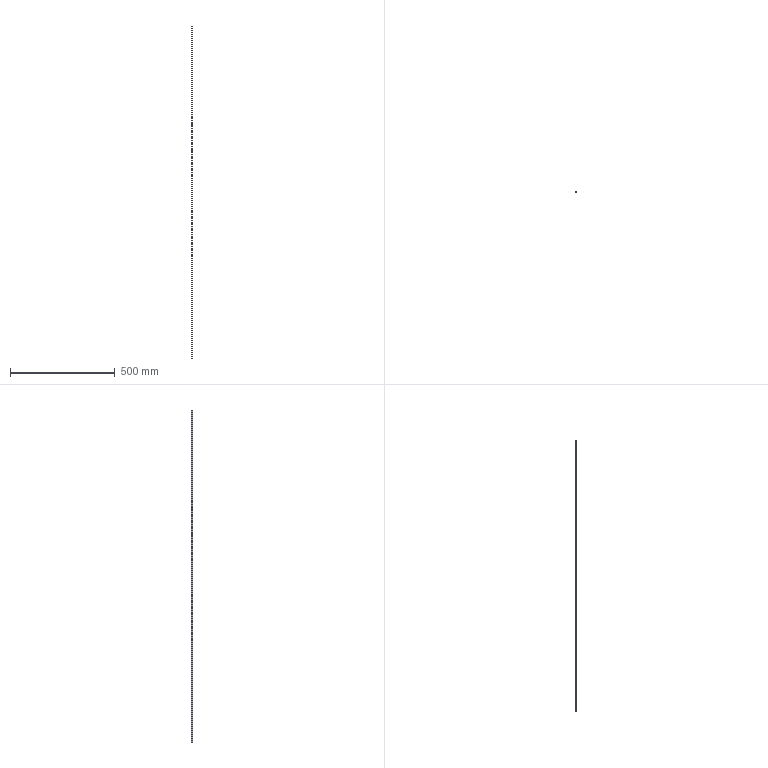Component | SolidWorks | D-SideAluminumHousingAssembly-1_D-SideSealant-1 | 1 solid | 6 faces | box 3 x 6 x 1582 mm | volume 28476 mm3 | plane 6
build123d program:
from build123d import *

# Parameters (mm, degrees)
SKETCH1_W           = 1582
SKETCH1_H           = 6
EXTRUDE_THIN1_DEPTH = 3


with BuildPart() as part:
    # Sketch1 → Extrude-Thin1 (new body)
    with BuildSketch(Plane.XY):
        with Locations((791, -3)):
            Rectangle(SKETCH1_W, SKETCH1_H)
    extrude(amount=EXTRUDE_THIN1_DEPTH)


solid = part.part

# Placed as in the assembly
solid = solid.moved(Location((-1015.5, 2312, 1728.5), (0, 90, 0)))
STEP:
#1=COLOUR_RGB('',0.7922,0.8196,0.9333);
#2=FILL_AREA_STYLE_COLOUR('',#1);
#3=FILL_AREA_STYLE('',(#2));
#4=SURFACE_STYLE_FILL_AREA(#3);
#5=SURFACE_SIDE_STYLE('',(#4));
#6=SURFACE_STYLE_USAGE(.BOTH.,#5);
#7=PRESENTATION_STYLE_ASSIGNMENT((#6));
#8=CARTESIAN_POINT('',(-39.862,90.787,5.768));
#9=VERTEX_POINT('',#8);
#10=CARTESIAN_POINT('',(-39.862,90.787,68.051));
#11=VERTEX_POINT('',#10);
#12=CARTESIAN_POINT('',(-39.862,90.787,5.768));
#13=DIRECTION('',(-0.,-0.,1.));
#14=VECTOR('',#13,39.37);
#15=LINE('',#12,#14);
#16=EDGE_CURVE('',#9,#11,#15,.T.);
#17=ORIENTED_EDGE('',*,*,#16,.T.);
#18=CARTESIAN_POINT('',(-39.98,90.787,68.051));
#19=VERTEX_POINT('',#18);
#20=CARTESIAN_POINT('',(-39.98,90.787,68.051));
#21=DIRECTION('',(1.,0.,0.));
#22=VECTOR('',#21,39.37);
#23=LINE('',#20,#22);
#24=EDGE_CURVE('',#19,#11,#23,.T.);
#25=ORIENTED_EDGE('',*,*,#24,.F.);
#26=CARTESIAN_POINT('',(-39.98,90.787,5.768));
#27=VERTEX_POINT('',#26);
#28=CARTESIAN_POINT('',(-39.98,90.787,5.768));
#29=DIRECTION('',(-0.,-0.,1.));
#30=VECTOR('',#29,39.37);
#31=LINE('',#28,#30);
#32=EDGE_CURVE('',#27,#19,#31,.T.);
#33=ORIENTED_EDGE('',*,*,#32,.F.);
#34=CARTESIAN_POINT('',(-39.98,90.787,5.768));
#35=DIRECTION('',(1.,0.,0.));
#36=VECTOR('',#35,39.37);
#37=LINE('',#34,#36);
#38=EDGE_CURVE('',#27,#9,#37,.T.);
#39=ORIENTED_EDGE('',*,*,#38,.T.);
#40=EDGE_LOOP('',(#17,#25,#33,#39));
#41=FACE_OUTER_BOUND('',#40,.T.);
#42=CARTESIAN_POINT('',(-39.98,90.787,5.768));
#43=DIRECTION('',(-0.,1.,0.));
#44=DIRECTION('',(-1.,-0.,-0.));
#45=AXIS2_PLACEMENT_3D('',#42,#43,#44);
#46=PLANE('',#45);
#47=ADVANCED_FACE('',(#41),#46,.F.);
#48=CARTESIAN_POINT('',(-39.862,91.024,68.051));
#49=VERTEX_POINT('',#48);
#50=CARTESIAN_POINT('',(-39.862,91.024,68.051));
#51=DIRECTION('',(0.,-1.,-0.));
#52=VECTOR('',#51,39.37);
#53=LINE('',#50,#52);
#54=EDGE_CURVE('',#49,#11,#53,.T.);
#55=ORIENTED_EDGE('',*,*,#54,.F.);
#56=CARTESIAN_POINT('',(-39.98,91.024,68.051));
#57=VERTEX_POINT('',#56);
#58=CARTESIAN_POINT('',(-39.98,91.024,68.051));
#59=DIRECTION('',(1.,0.,0.));
#60=VECTOR('',#59,39.37);
#61=LINE('',#58,#60);
#62=EDGE_CURVE('',#57,#49,#61,.T.);
#63=ORIENTED_EDGE('',*,*,#62,.F.);
#64=CARTESIAN_POINT('',(-39.98,91.024,68.051));
#65=DIRECTION('',(0.,-1.,-0.));
#66=VECTOR('',#65,39.37);
#67=LINE('',#64,#66);
#68=EDGE_CURVE('',#57,#19,#67,.T.);
#69=ORIENTED_EDGE('',*,*,#68,.T.);
#70=ORIENTED_EDGE('',*,*,#24,.T.);
#71=EDGE_LOOP('',(#55,#63,#69,#70));
#72=FACE_OUTER_BOUND('',#71,.T.);
#73=CARTESIAN_POINT('',(-39.98,91.024,68.051));
#74=DIRECTION('',(-0.,-0.,1.));
#75=DIRECTION('',(1.,0.,0.));
#76=AXIS2_PLACEMENT_3D('',#73,#74,#75);
#77=PLANE('',#76);
#78=ADVANCED_FACE('',(#72),#77,.T.);
#79=CARTESIAN_POINT('',(-39.862,91.024,5.768));
#80=VERTEX_POINT('',#79);
#81=CARTESIAN_POINT('',(-39.862,91.024,5.768));
#82=DIRECTION('',(-0.,-0.,1.));
#83=VECTOR('',#82,39.37);
#84=LINE('',#81,#83);
#85=EDGE_CURVE('',#80,#49,#84,.T.);
#86=ORIENTED_EDGE('',*,*,#85,.F.);
#87=CARTESIAN_POINT('',(-39.98,91.024,5.768));
#88=VERTEX_POINT('',#87);
#89=CARTESIAN_POINT('',(-39.98,91.024,5.768));
#90=DIRECTION('',(1.,0.,0.));
#91=VECTOR('',#90,39.37);
#92=LINE('',#89,#91);
#93=EDGE_CURVE('',#88,#80,#92,.T.);
#94=ORIENTED_EDGE('',*,*,#93,.F.);
#95=CARTESIAN_POINT('',(-39.98,91.024,5.768));
#96=DIRECTION('',(-0.,-0.,1.));
#97=VECTOR('',#96,39.37);
#98=LINE('',#95,#97);
#99=EDGE_CURVE('',#88,#57,#98,.T.);
#100=ORIENTED_EDGE('',*,*,#99,.T.);
#101=ORIENTED_EDGE('',*,*,#62,.T.);
#102=EDGE_LOOP('',(#86,#94,#100,#101));
#103=FACE_OUTER_BOUND('',#102,.T.);
#104=CARTESIAN_POINT('',(-39.98,91.024,5.768));
#105=DIRECTION('',(-0.,1.,0.));
#106=DIRECTION('',(-1.,-0.,-0.));
#107=AXIS2_PLACEMENT_3D('',#104,#105,#106);
#108=PLANE('',#107);
#109=ADVANCED_FACE('',(#103),#108,.T.);
#110=CARTESIAN_POINT('',(-39.862,90.787,5.768));
#111=DIRECTION('',(-0.,1.,0.));
#112=VECTOR('',#111,39.37);
#113=LINE('',#110,#112);
#114=EDGE_CURVE('',#9,#80,#113,.T.);
#115=ORIENTED_EDGE('',*,*,#114,.F.);
#116=ORIENTED_EDGE('',*,*,#38,.F.);
#117=CARTESIAN_POINT('',(-39.98,90.787,5.768));
#118=DIRECTION('',(-0.,1.,0.));
#119=VECTOR('',#118,39.37);
#120=LINE('',#117,#119);
#121=EDGE_CURVE('',#27,#88,#120,.T.);
#122=ORIENTED_EDGE('',*,*,#121,.T.);
#123=ORIENTED_EDGE('',*,*,#93,.T.);
#124=EDGE_LOOP('',(#115,#116,#122,#123));
#125=FACE_OUTER_BOUND('',#124,.T.);
#126=CARTESIAN_POINT('',(-39.98,90.787,5.768));
#127=DIRECTION('',(0.,0.,-1.));
#128=DIRECTION('',(-1.,-0.,-0.));
#129=AXIS2_PLACEMENT_3D('',#126,#127,#128);
#130=PLANE('',#129);
#131=ADVANCED_FACE('',(#125),#130,.T.);
#132=ORIENTED_EDGE('',*,*,#32,.T.);
#133=ORIENTED_EDGE('',*,*,#68,.F.);
#134=ORIENTED_EDGE('',*,*,#99,.F.);
#135=ORIENTED_EDGE('',*,*,#121,.F.);
#136=EDGE_LOOP('',(#132,#133,#134,#135));
#137=FACE_OUTER_BOUND('',#136,.T.);
#138=CARTESIAN_POINT('',(-39.98,91.024,5.768));
#139=DIRECTION('',(1.,0.,0.));
#140=DIRECTION('',(0.,0.,-1.));
#141=AXIS2_PLACEMENT_3D('',#138,#139,#140);
#142=PLANE('',#141);
#143=ADVANCED_FACE('',(#137),#142,.F.);
#144=ORIENTED_EDGE('',*,*,#16,.F.);
#145=ORIENTED_EDGE('',*,*,#114,.T.);
#146=ORIENTED_EDGE('',*,*,#85,.T.);
#147=ORIENTED_EDGE('',*,*,#54,.T.);
#148=EDGE_LOOP('',(#144,#145,#146,#147));
#149=FACE_OUTER_BOUND('',#148,.T.);
#150=CARTESIAN_POINT('',(-39.862,91.024,5.768));
#151=DIRECTION('',(1.,0.,0.));
#152=DIRECTION('',(0.,0.,-1.));
#153=AXIS2_PLACEMENT_3D('',#150,#151,#152);
#154=PLANE('',#153);
#155=ADVANCED_FACE('',(#149),#154,.T.);
#156=CLOSED_SHELL('',(#47,#78,#109,#131,#143,#155));
#157=MANIFOLD_SOLID_BREP('',#156);
#158=STYLED_ITEM('',(#7),#157);
#159=PRESENTATION_LAYER_ASSIGNMENT('','',(#158));
#160=(LENGTH_UNIT()NAMED_UNIT(*)SI_UNIT($,.METRE.));
#161=LENGTH_MEASURE_WITH_UNIT(LENGTH_MEASURE(0.0254),#160);
#162=DIMENSIONAL_EXPONENTS(1.,0.,0.,0.,0.,0.,0.);
#163=(CONVERSION_BASED_UNIT('',#161)LENGTH_UNIT()NAMED_UNIT(#162));
#164=UNCERTAINTY_MEASURE_WITH_UNIT(LENGTH_MEASURE(0.00001),#163,'','');
#165=(NAMED_UNIT(*)PLANE_ANGLE_UNIT()SI_UNIT($,.RADIAN.));
#166=(NAMED_UNIT(*)SI_UNIT($,.STERADIAN.)SOLID_ANGLE_UNIT());
#167=(GEOMETRIC_REPRESENTATION_CONTEXT(3)GLOBAL_UNCERTAINTY_ASSIGNED_CONTEXT((#164))GLOBAL_UNIT_ASSIGNED_CONTEXT((#163,#165,#166))REPRESENTATION_CONTEXT('',''));
#168=MECHANICAL_DESIGN_GEOMETRIC_PRESENTATION_REPRESENTATION('',(#158),#167);
#169=CARTESIAN_POINT('',(0.,0.,0.));
#170=DIRECTION('',(0.,0.,1.));
#171=DIRECTION('',(1.,0.,0.));
#172=AXIS2_PLACEMENT_3D('',#169,#170,#171);
#173=(LENGTH_UNIT()NAMED_UNIT(*)SI_UNIT($,.METRE.));
#174=LENGTH_MEASURE_WITH_UNIT(LENGTH_MEASURE(0.0254),#173);
#175=DIMENSIONAL_EXPONENTS(1.,0.,0.,0.,0.,0.,0.);
#176=(CONVERSION_BASED_UNIT('',#174)LENGTH_UNIT()NAMED_UNIT(#175));
#177=UNCERTAINTY_MEASURE_WITH_UNIT(LENGTH_MEASURE(0.00001),#176,'','');
#178=(NAMED_UNIT(*)PLANE_ANGLE_UNIT()SI_UNIT($,.RADIAN.));
#179=(NAMED_UNIT(*)SI_UNIT($,.STERADIAN.)SOLID_ANGLE_UNIT());
#180=(GEOMETRIC_REPRESENTATION_CONTEXT(3)GLOBAL_UNCERTAINTY_ASSIGNED_CONTEXT((#177))GLOBAL_UNIT_ASSIGNED_CONTEXT((#176,#178,#179))REPRESENTATION_CONTEXT('',''));
#181=ADVANCED_BREP_SHAPE_REPRESENTATION('',(#157,#172),#180);